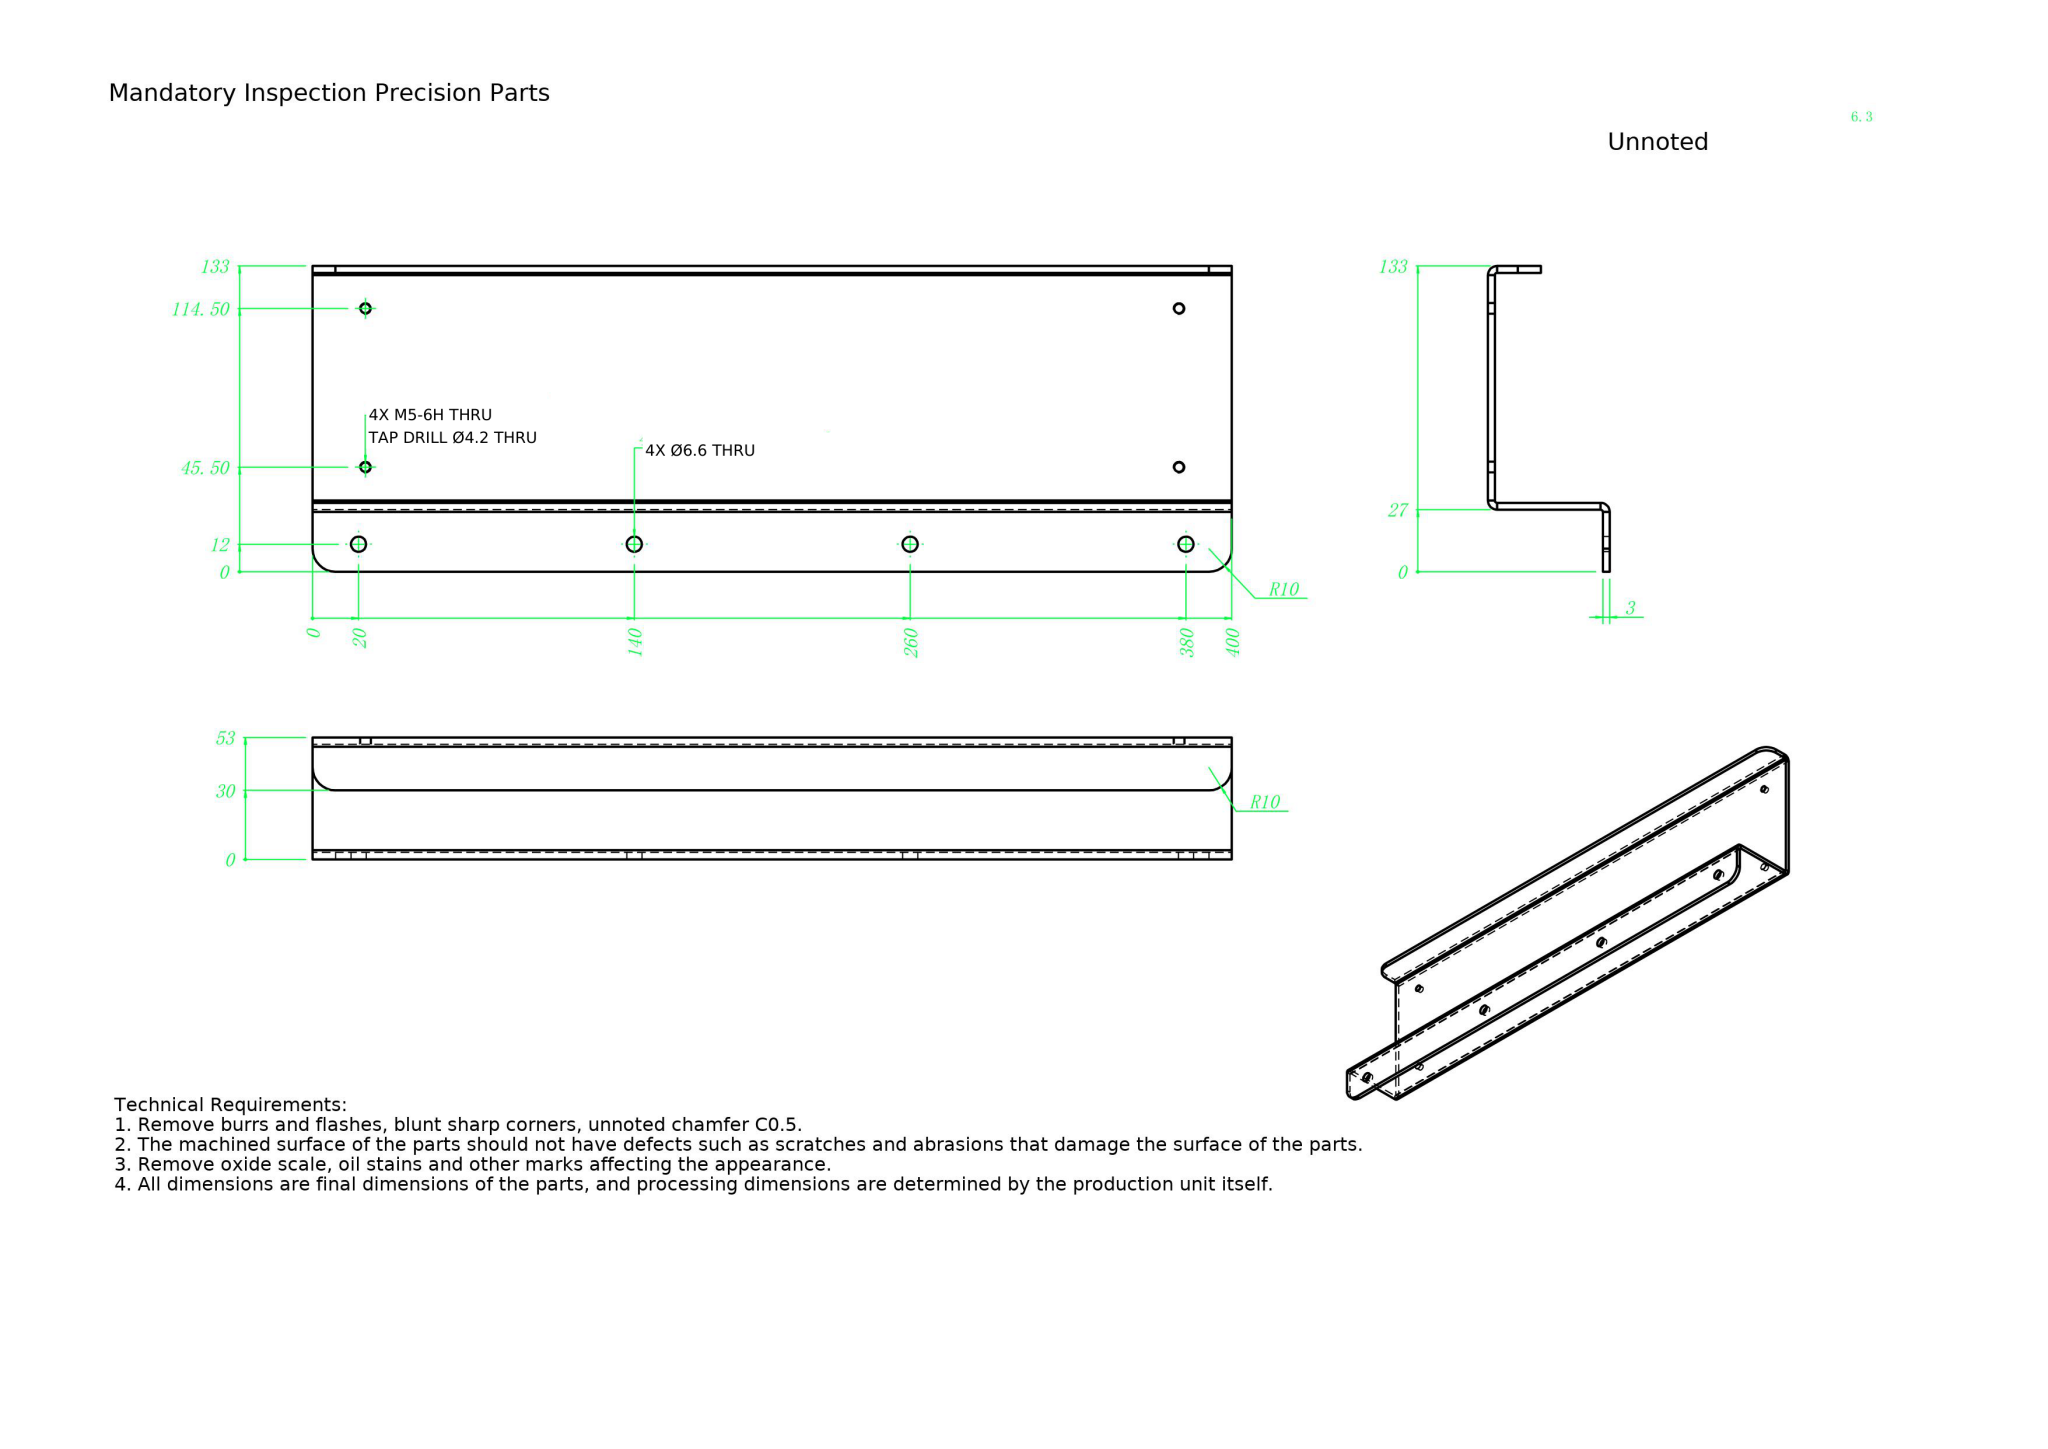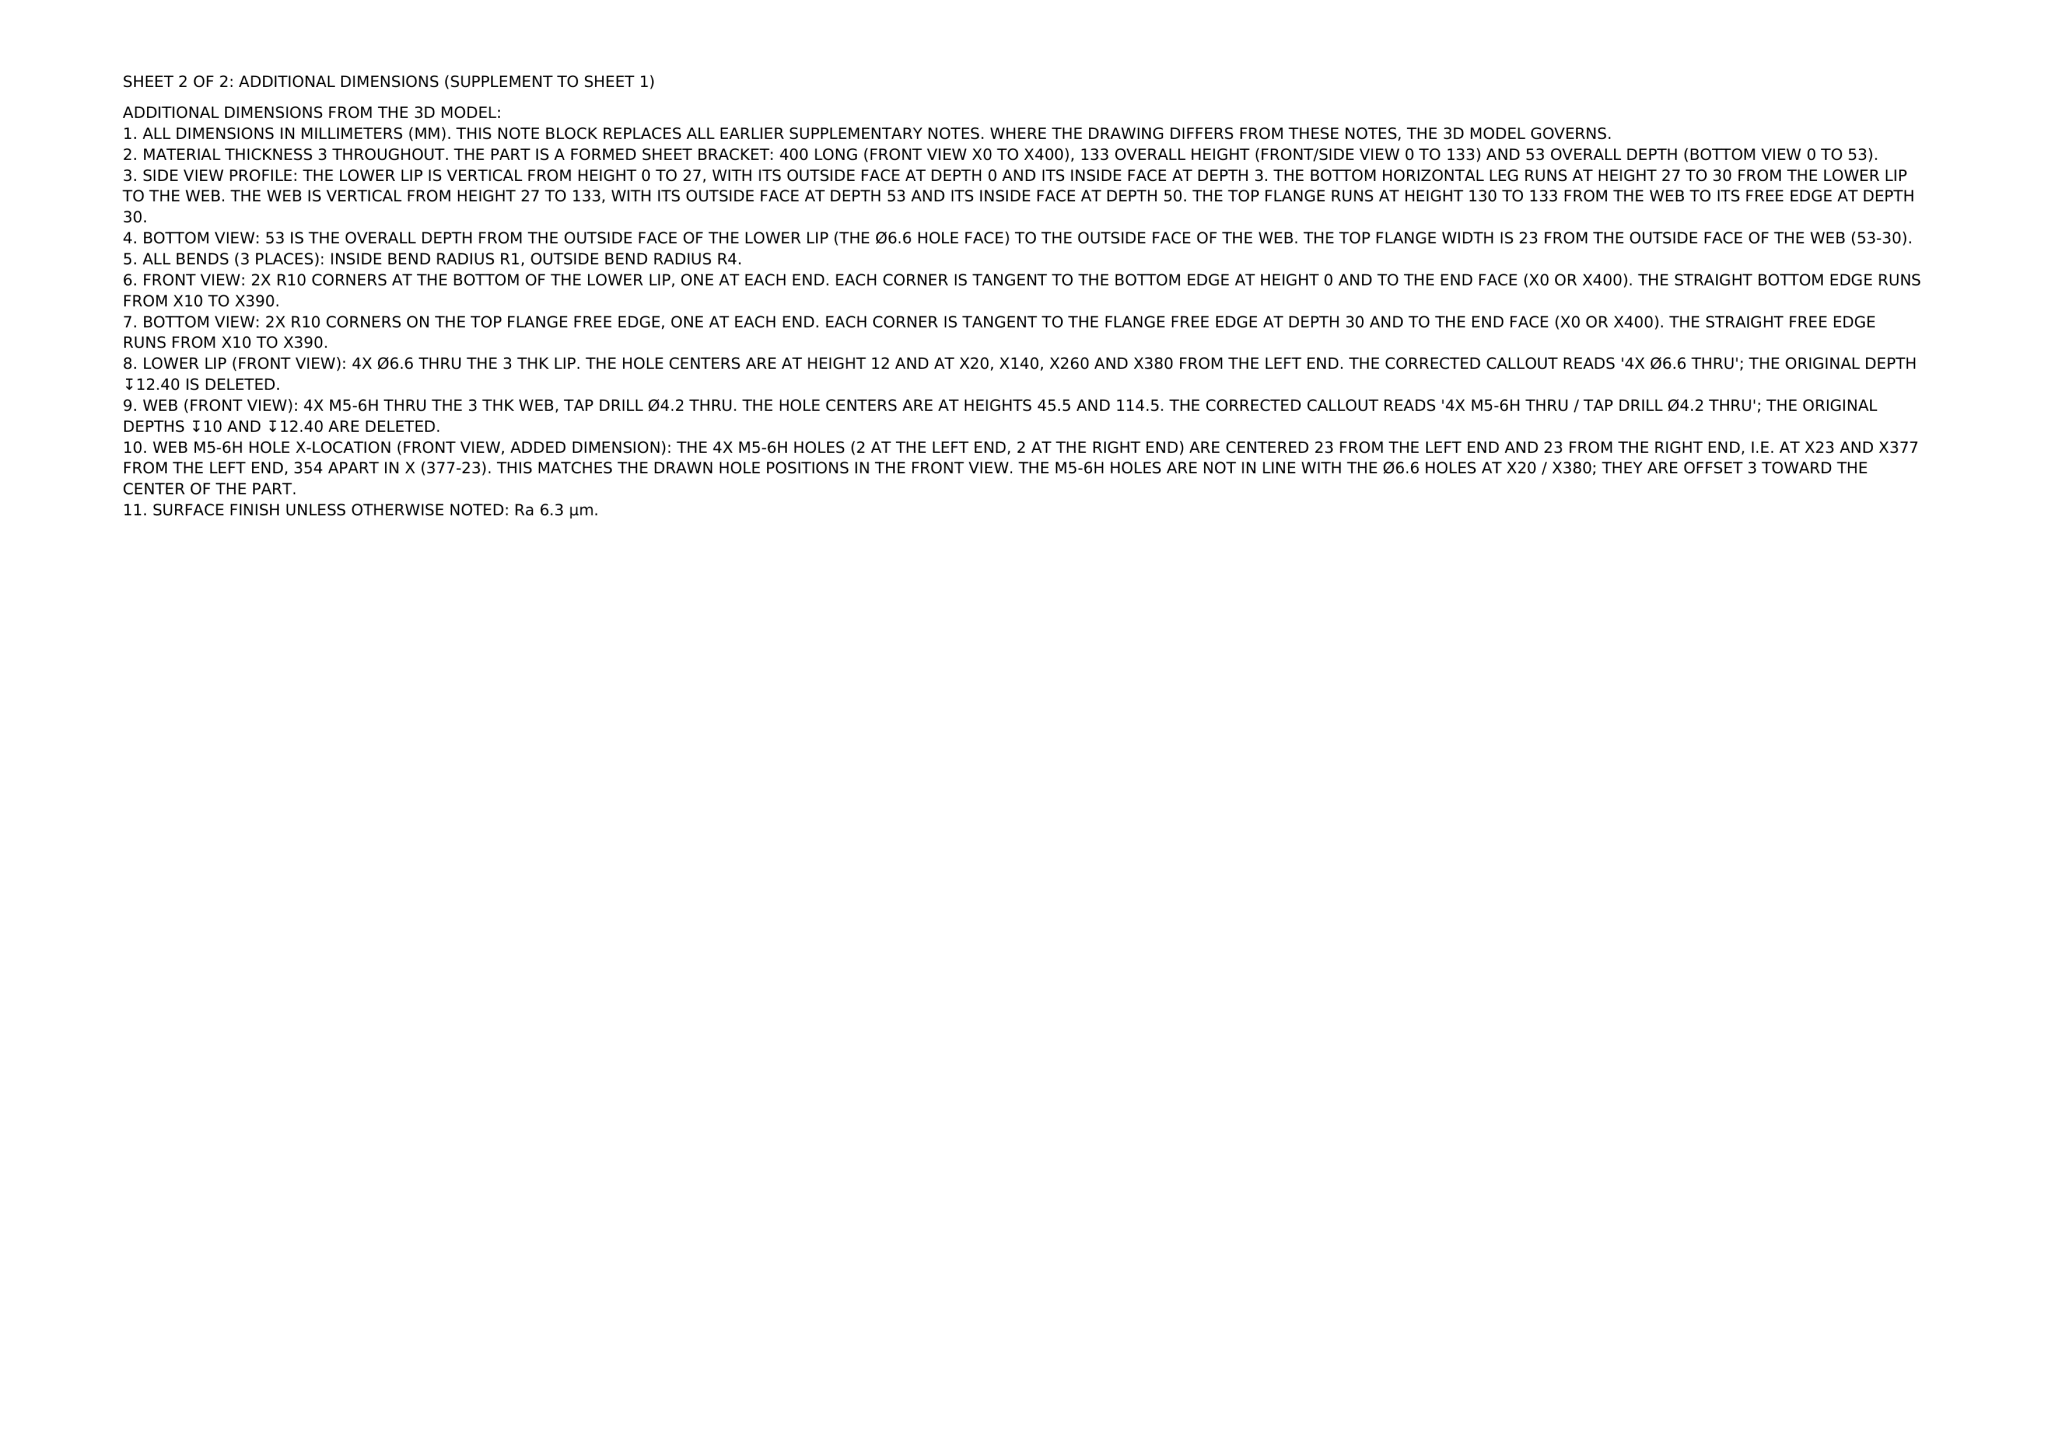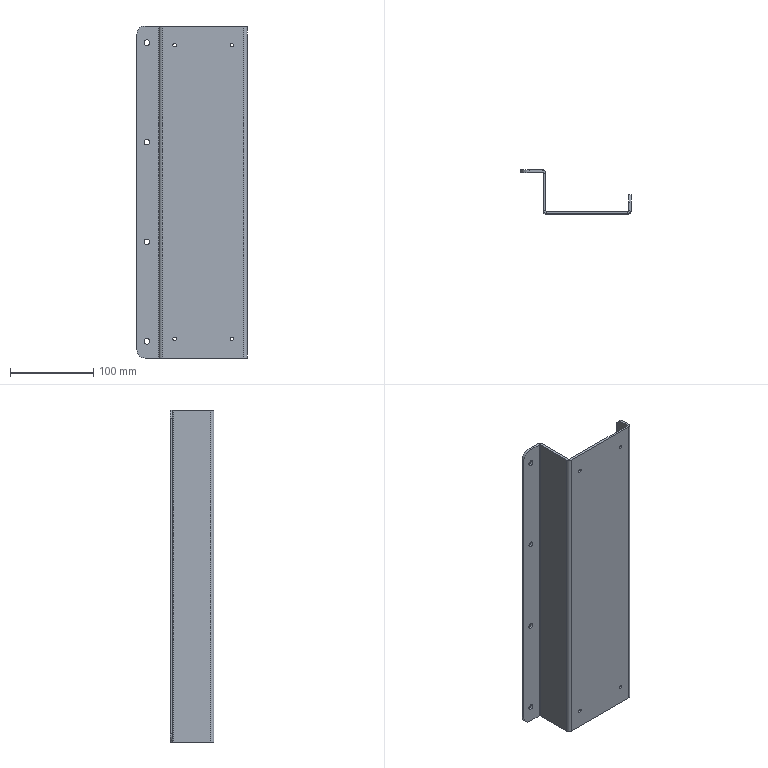Part | NX | mm | 1 solid | 50 faces | box 133 x 53 x 400 mm | volume 238903 mm3 | cylinder 26 | plane 24 | commonest cylinder face diameters 6.6 x8 4.2 x8 20 x4 2 x3 8 x3